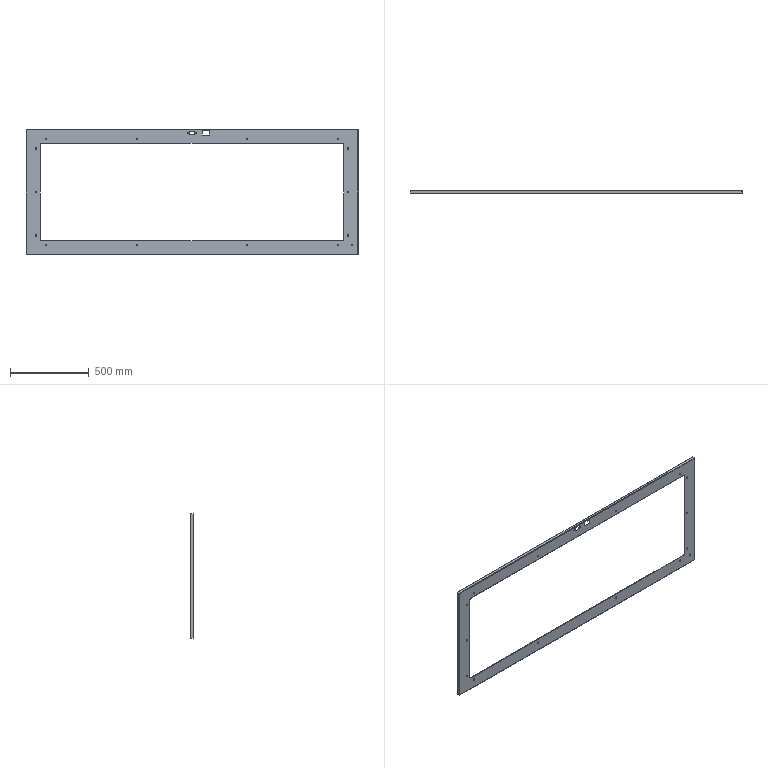Component | SolidWorks | FrontDoorAssembly-1_FrontDoorWelding-1_FrontDoorFrame(Riveted)PG50-02-101-1_FrontDoorFramePG50-02-101-1 | 1 solid | 151 faces | volume 1133852 mm3 | cylinder 84 | plane 67 | commonest cylinder face diameters 9.3 x30 6 x30 12 x8 8.5 x4 20 x4 4.3 x4 0.3 x4 | material AISI 1045 Steel, cold drawn